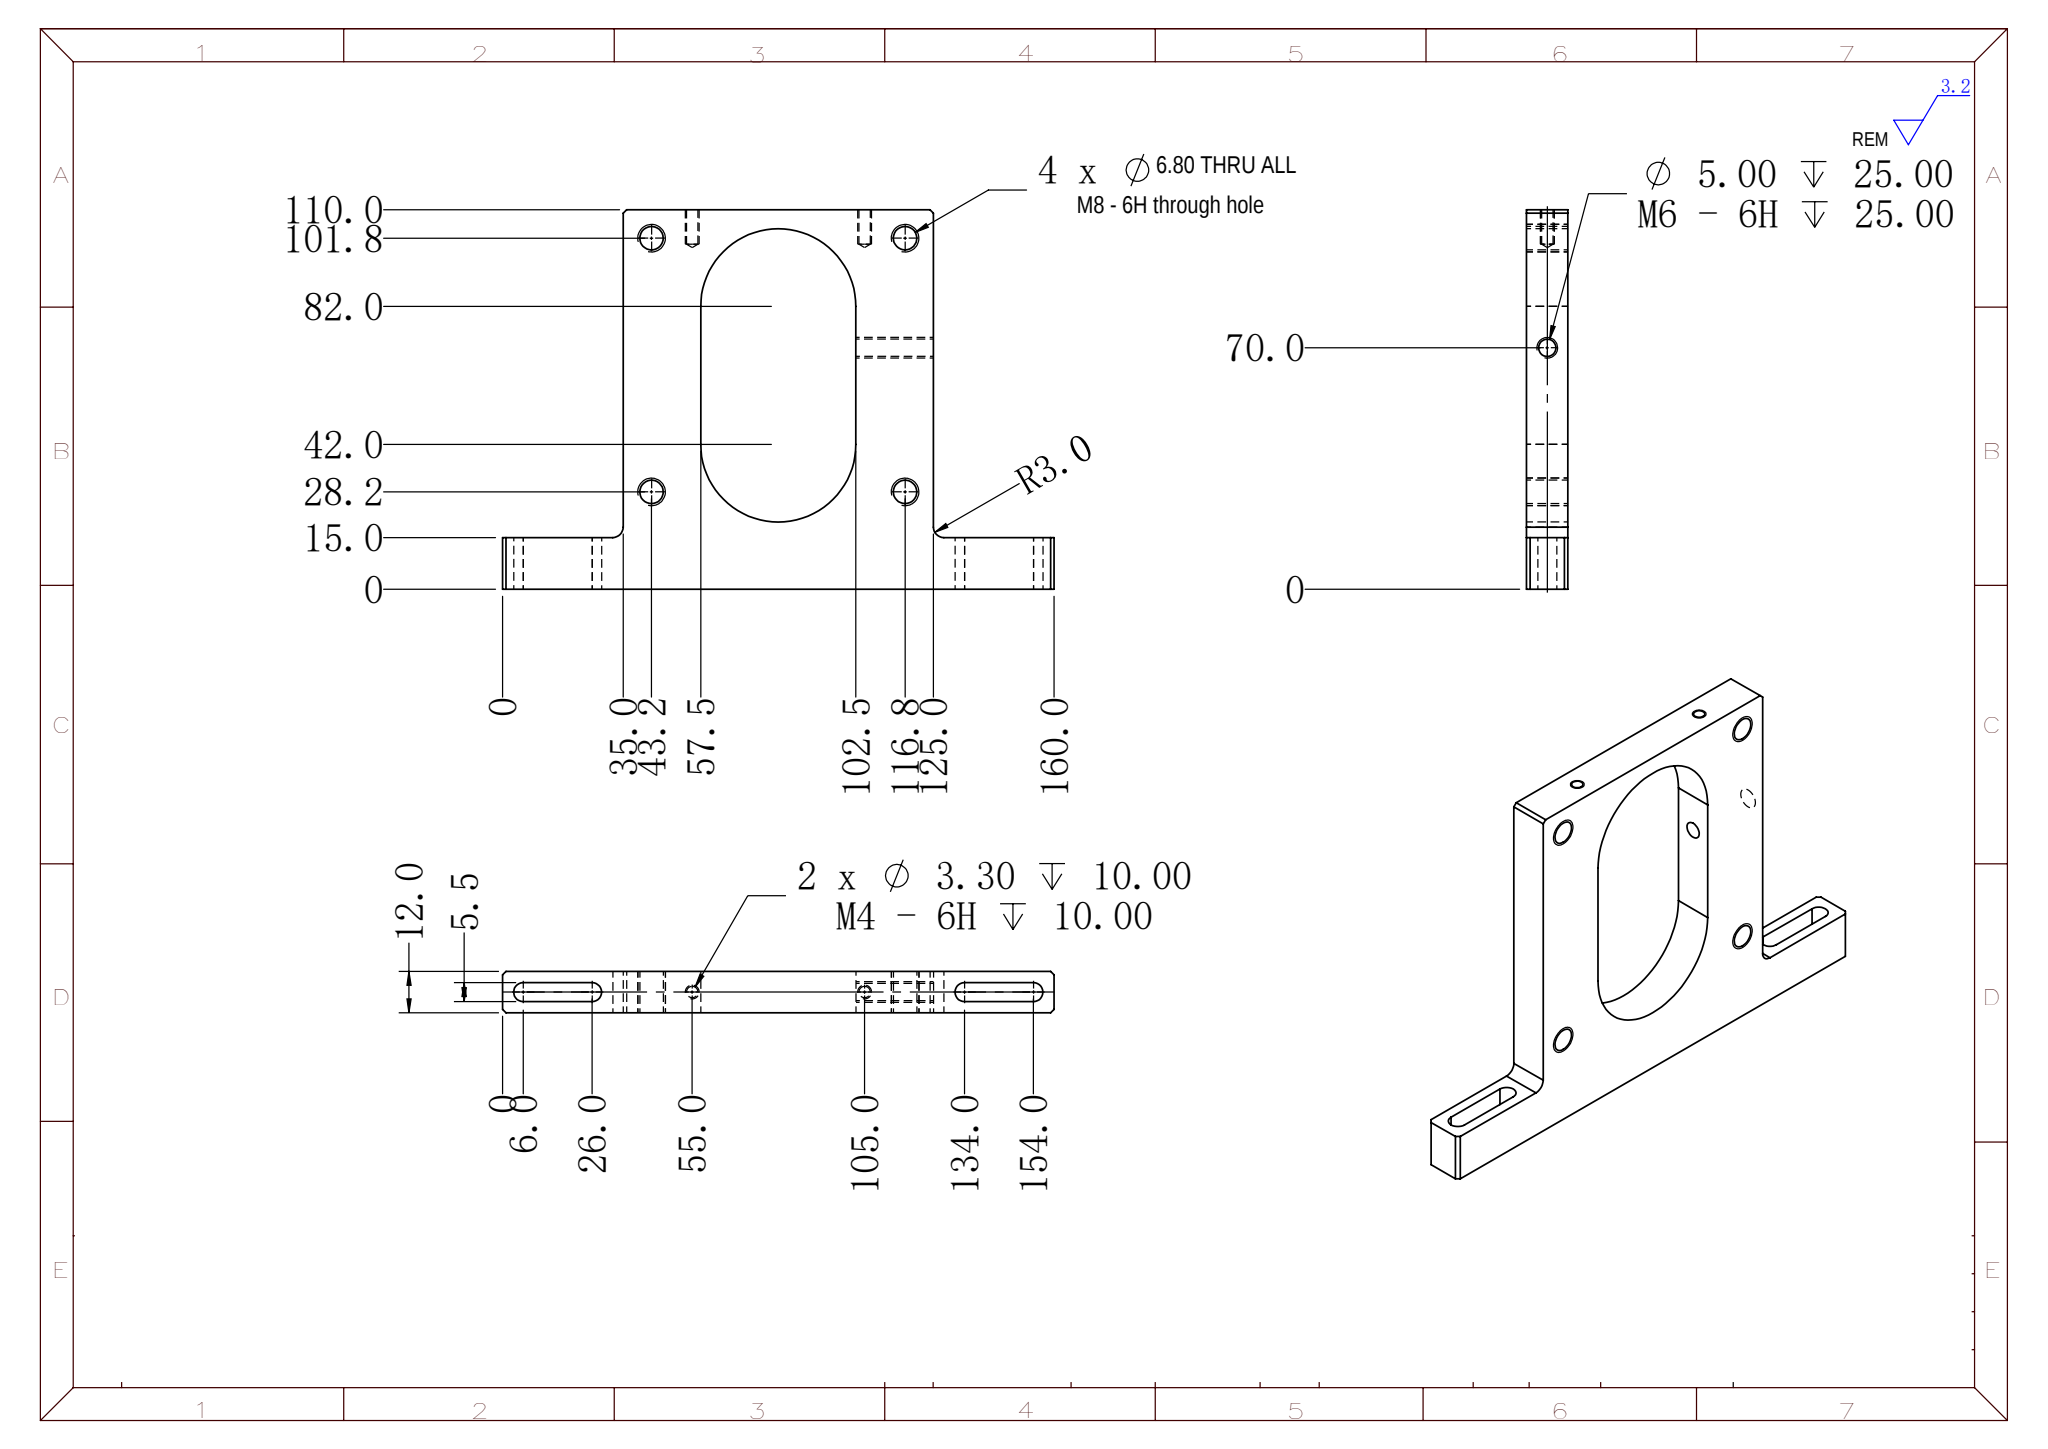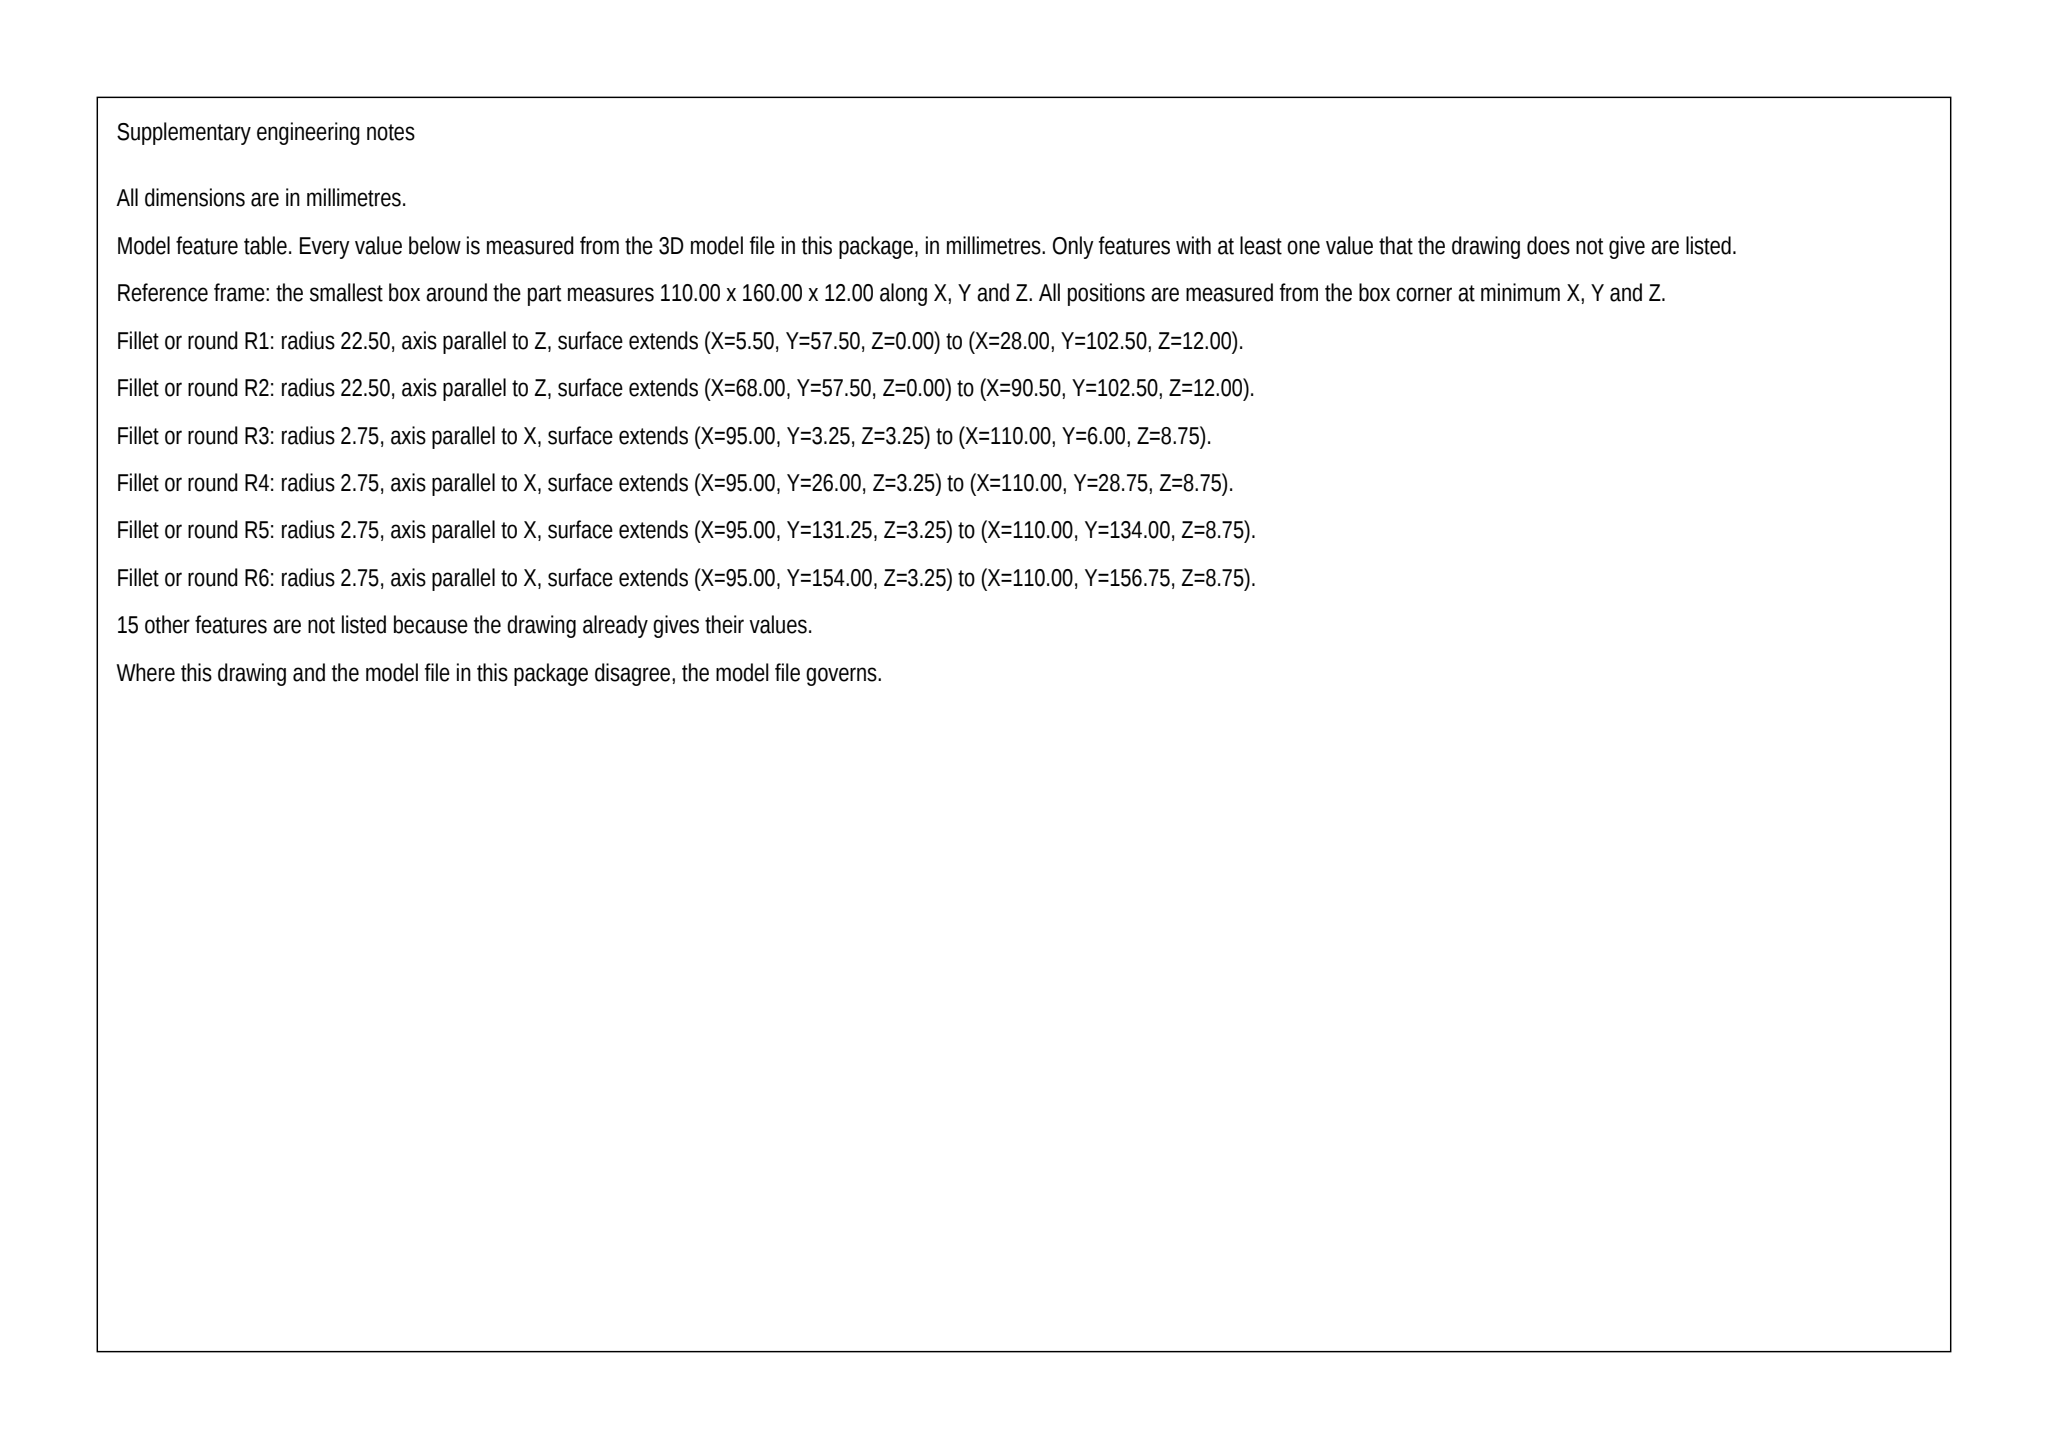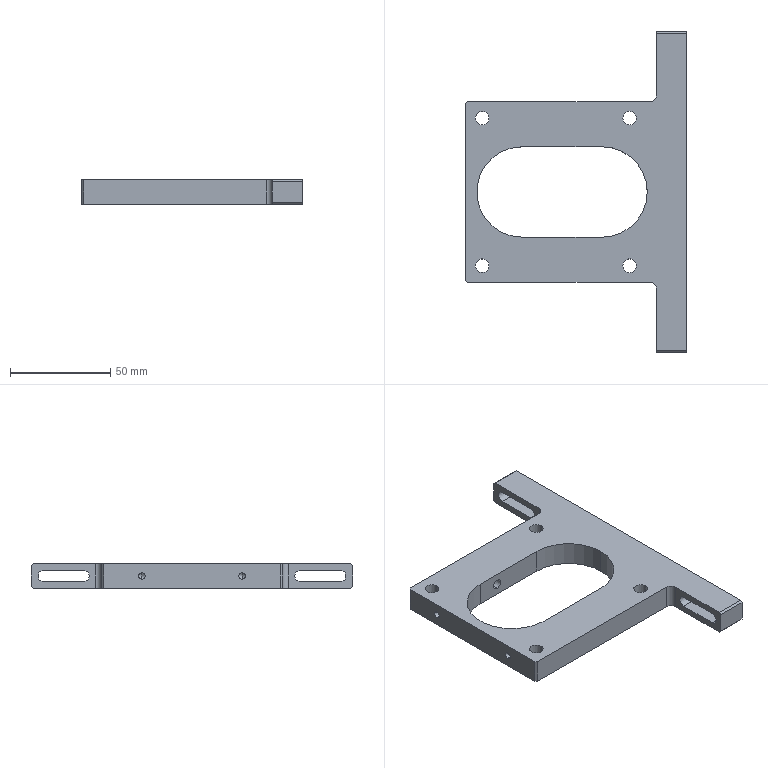Part | SolidWorks | mm | 1 solid | 49 faces | box 110 x 160 x 12 mm | volume 84345 mm3 | cylinder 23 | plane 22 | cone 4 | commonest cylinder face diameters 6.8 x8 3.3 x4 5.5 x4 45 x3 5 x2 6 x2
build123d program:
from build123d import *

# Parameters (mm, degrees)
SKETCH1_W             = 110
SKETCH1_H             = 90
BOSS_EXTRUDE1_DEPTH   = 6
CUT_EXTRUDE1_DEPTH    = 73.069
M8_TAPPED_HOLE1_D     = 6.8
M6_TAPPED_HOLE1_D     = 5
M6_TAPPED_HOLE1_DEPTH = 25
M6_TAPPED_HOLE1_TIP   = 1.502
SKETCH12_W            = 15
SKETCH12_H            = 35
BOSS_EXTRUDE2_DEPTH   = 12
CUT_EXTRUDE5_DEPTH    = 125.342
FILLET1_R             = 3
M4_TAPPED_HOLE1_D     = 3.3
M4_TAPPED_HOLE1_DEPTH = 10
M4_TAPPED_HOLE1_TIP   = 0.9914
CHAMFER1_SIZE         = 1


with BuildPart() as part:
    # Sketch1 → Boss-Extrude1 (new, symmetric)
    with BuildSketch(Plane.XY):
        Rectangle(SKETCH1_W, SKETCH1_H)
    extrude(amount=BOSS_EXTRUDE1_DEPTH, both=True)

    # Sketch2 → Cut-Extrude1 (cut, through all)
    with BuildSketch(Plane.XY.offset(6)):
        with BuildLine():
            Line((-27, 22.5), (13, 22.5))
            ThreePointArc((13, 22.5), (35.5, 0), (13, -22.5))
            Line((13, -22.5), (-27, -22.5))
            ThreePointArc((-27, -22.5), (-49.5, 0), (-27, 22.5))
        make_face()
    extrude(amount=-CUT_EXTRUDE1_DEPTH, mode=Mode.SUBTRACT)

    # M8 Tapped Hole1 (through all)
    with Locations(Plane.XY.offset(6)):
        with Locations((-46.77, 36.77), (-46.77, -36.77), (26.77, -36.77), (26.77, 36.77)):
            Hole(M8_TAPPED_HOLE1_D / 2)

    # M6 Tapped Hole1
    with Locations(Plane(origin=(0, 45, 0), x_dir=(1, 0, 0), z_dir=(0, 1, 0))):
        with Locations((-15, 0)):
            Hole(M6_TAPPED_HOLE1_D / 2, depth=M6_TAPPED_HOLE1_DEPTH)
            with Locations((0, 0, -(M6_TAPPED_HOLE1_DEPTH + M6_TAPPED_HOLE1_TIP / 2))):  # 118° drill point
                Cone(0, M6_TAPPED_HOLE1_D / 2, M6_TAPPED_HOLE1_TIP, mode=Mode.SUBTRACT)

    # Sketch12 → Boss-Extrude2 (add)
    with BuildSketch(Plane.XY.offset(6)):
        with Locations((47.5, -62.5)):
            Rectangle(SKETCH12_W, SKETCH12_H)
        with Locations((47.5, 62.5)):
            Rectangle(SKETCH12_W, SKETCH12_H)
    extrude(amount=-BOSS_EXTRUDE2_DEPTH)

    # Sketch13 → Cut-Extrude5 (cut, through all)
    with BuildSketch(Plane.ZY.offset(-40)):
        with BuildLine():
            Line((-2.75, -74), (-2.75, -54))
            ThreePointArc((-2.75, -54), (0, -51.25), (2.75, -54))
            Line((2.75, -54), (2.75, -74))
            ThreePointArc((2.75, -74), (0, -76.75), (-2.75, -74))
        make_face()
        with BuildLine():
            Line((-2.75, 74), (-2.75, 54))
            ThreePointArc((-2.75, 54), (0, 51.25), (2.75, 54))
            Line((2.75, 54), (2.75, 74))
            ThreePointArc((2.75, 74), (0, 76.75), (-2.75, 74))
        make_face()
    extrude(amount=-CUT_EXTRUDE5_DEPTH, mode=Mode.SUBTRACT)

    # Fillet1
    fillet1_edges = [part.edges().sort_by_distance(p)[0] for p in [
        (40, -45, 0),
        (40, 45, 0),
    ]]
    fillet(fillet1_edges, radius=FILLET1_R)

    # M4 Tapped Hole1
    with Locations(Plane.ZY.offset(55)):
        with Locations((0, -25), (0, 25)):
            Hole(M4_TAPPED_HOLE1_D / 2, depth=M4_TAPPED_HOLE1_DEPTH)
            with Locations((0, 0, -(M4_TAPPED_HOLE1_DEPTH + M4_TAPPED_HOLE1_TIP / 2))):  # 118° drill point
                Cone(0, M4_TAPPED_HOLE1_D / 2, M4_TAPPED_HOLE1_TIP, mode=Mode.SUBTRACT)

    # Chamfer1
    chamfer1_edges = [part.edges().sort_by_distance(p)[0] for p in [
        (47.5, -80, 6),
        (47.5, -80, -6),
        (47.5, 80, 6),
        (47.5, 80, -6),
        (-55, -45, 0),
        (-55, 45, 0),
    ]]
    chamfer(chamfer1_edges, length=CHAMFER1_SIZE)


solid = part.part